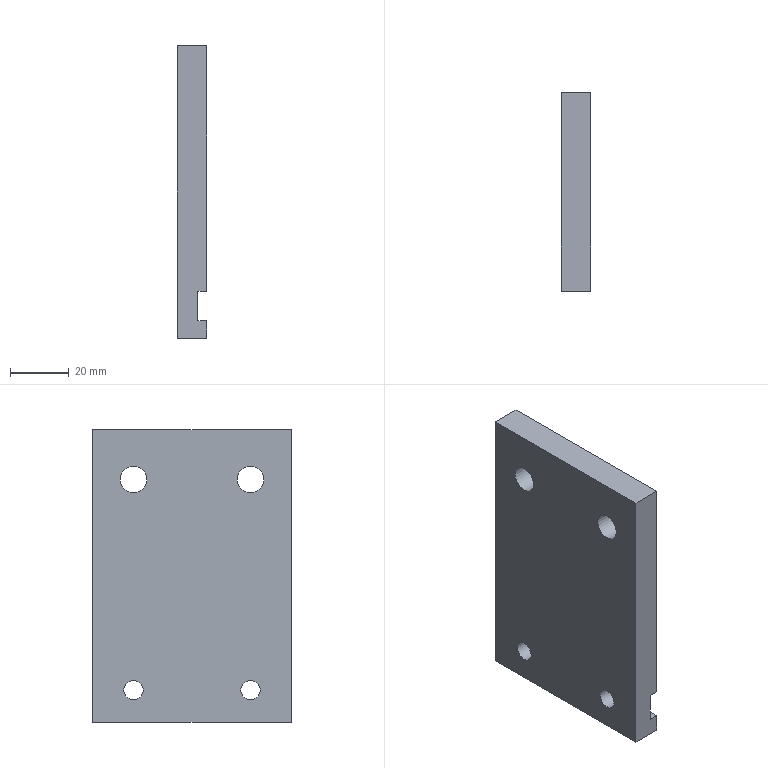Component | NX | GRIPPER_JAW_2 | 1 solid | 14 faces | box 10 x 68 x 100 mm | volume 64209 mm3 | plane 10 | cylinder 4 | commonest cylinder face diameters 6.6 x2 9 x2
STEP:
#1=CARTESIAN_POINT('',(0.,0.,0.));
#2=DIRECTION('',(0.,0.,1.));
#3=DIRECTION('',(1.,0.,0.));
#4=AXIS2_PLACEMENT_3D('',#1,#2,#3);
#5=CARTESIAN_POINT('',(-23.5,223.462,123.766));
#6=VERTEX_POINT('',#5);
#7=CARTESIAN_POINT('',(-23.5,223.462,120.466));
#8=DIRECTION('',(1.,0.,0.));
#9=DIRECTION('',(0.,0.,1.));
#10=AXIS2_PLACEMENT_3D('',#7,#8,#9);
#11=CIRCLE('',#10,3.3);
#12=CARTESIAN_POINT('',(-23.5,223.462,120.466));
#13=DIRECTION('',(1.,0.,0.));
#14=DIRECTION('',(0.,0.,-1.));
#15=AXIS2_PLACEMENT_3D('',#12,#13,#14);
#16=CYLINDRICAL_SURFACE('',#15,3.3);
#17=CARTESIAN_POINT('',(3.142,0.));
#18=DIRECTION('',(1.,0.));
#19=VECTOR('',#18,1.);
#20=LINE('',#17,#19);
#21=(GEOMETRIC_REPRESENTATION_CONTEXT(2)PARAMETRIC_REPRESENTATION_CONTEXT()REPRESENTATION_CONTEXT('',''));
#22=DEFINITIONAL_REPRESENTATION('',(#20),#21);
#23=PCURVE('',#16,#22);
#24=CARTESIAN_POINT('',(-23.5,223.462,192.466));
#25=DIRECTION('',(1.,0.,0.));
#26=DIRECTION('',(0.,0.,-1.));
#27=AXIS2_PLACEMENT_3D('',#24,#25,#26);
#28=PLANE('',#27);
#29=CARTESIAN_POINT('',(72.,0.));
#30=DIRECTION('',(-1.,0.));
#31=AXIS2_PLACEMENT_2D('',#29,#30);
#32=CIRCLE('',#31,3.3);
#33=(GEOMETRIC_REPRESENTATION_CONTEXT(2)PARAMETRIC_REPRESENTATION_CONTEXT()REPRESENTATION_CONTEXT('',''));
#34=DEFINITIONAL_REPRESENTATION('',(#32),#33);
#35=PCURVE('',#28,#34);
#36=SURFACE_CURVE('',#11,(#23,#35),.PCURVE_S1.);
#37=EDGE_CURVE('',#6,#6,#36,.T.);
#38=ORIENTED_EDGE('',*,*,#37,.T.);
#39=CARTESIAN_POINT('',(-16.5,223.462,123.766));
#40=VERTEX_POINT('',#39);
#41=CARTESIAN_POINT('',(-23.5,223.462,123.766));
#42=CARTESIAN_POINT('',(-16.5,223.462,123.766));
#43=B_SPLINE_CURVE_WITH_KNOTS('',1,(#41,#42),.UNSPECIFIED.,.F.,.F.,(2,2),(0.,7.),.PIECEWISE_BEZIER_KNOTS.);
#44=CARTESIAN_POINT('',(9.425,0.));
#45=DIRECTION('',(0.,1.));
#46=VECTOR('',#45,1.);
#47=LINE('',#44,#46);
#48=(GEOMETRIC_REPRESENTATION_CONTEXT(2)PARAMETRIC_REPRESENTATION_CONTEXT()REPRESENTATION_CONTEXT('',''));
#49=DEFINITIONAL_REPRESENTATION('',(#47),#48);
#50=PCURVE('',#16,#49);
#51=CARTESIAN_POINT('',(3.142,0.));
#52=DIRECTION('',(0.,1.));
#53=VECTOR('',#52,1.);
#54=LINE('',#51,#53);
#55=(GEOMETRIC_REPRESENTATION_CONTEXT(2)PARAMETRIC_REPRESENTATION_CONTEXT()REPRESENTATION_CONTEXT('',''));
#56=DEFINITIONAL_REPRESENTATION('',(#54),#55);
#57=PCURVE('',#16,#56);
#58=SEAM_CURVE('',#43,(#50,#57),.PCURVE_S1.);
#59=EDGE_CURVE('',#6,#40,#58,.T.);
#60=ORIENTED_EDGE('',*,*,#59,.T.);
#61=CARTESIAN_POINT('',(-16.5,223.462,120.466));
#62=DIRECTION('',(-1.,0.,0.));
#63=DIRECTION('',(0.,0.,1.));
#64=AXIS2_PLACEMENT_3D('',#61,#62,#63);
#65=CIRCLE('',#64,3.3);
#66=CARTESIAN_POINT('',(9.425,7.));
#67=DIRECTION('',(-1.,0.));
#68=VECTOR('',#67,1.);
#69=LINE('',#66,#68);
#70=(GEOMETRIC_REPRESENTATION_CONTEXT(2)PARAMETRIC_REPRESENTATION_CONTEXT()REPRESENTATION_CONTEXT('',''));
#71=DEFINITIONAL_REPRESENTATION('',(#69),#70);
#72=PCURVE('',#16,#71);
#73=CARTESIAN_POINT('',(-16.5,263.462,120.466));
#74=DIRECTION('',(-1.,0.,0.));
#75=DIRECTION('',(0.,0.,1.));
#76=AXIS2_PLACEMENT_3D('',#73,#74,#75);
#77=PLANE('',#76);
#78=CARTESIAN_POINT('',(0.,-40.));
#79=DIRECTION('',(1.,0.));
#80=AXIS2_PLACEMENT_2D('',#78,#79);
#81=CIRCLE('',#80,3.3);
#82=(GEOMETRIC_REPRESENTATION_CONTEXT(2)PARAMETRIC_REPRESENTATION_CONTEXT()REPRESENTATION_CONTEXT('',''));
#83=DEFINITIONAL_REPRESENTATION('',(#81),#82);
#84=PCURVE('',#77,#83);
#85=SURFACE_CURVE('',#65,(#72,#84),.PCURVE_S1.);
#86=EDGE_CURVE('',#40,#40,#85,.T.);
#87=ORIENTED_EDGE('',*,*,#86,.T.);
#88=ORIENTED_EDGE('',*,*,#59,.F.);
#89=EDGE_LOOP('',(#38,#60,#87,#88));
#90=FACE_BOUND('',#89,.F.);
#91=ADVANCED_FACE('',(#90),#16,.F.);
#92=CARTESIAN_POINT('',(-13.5,209.462,115.466));
#93=VERTEX_POINT('',#92);
#94=CARTESIAN_POINT('',(-13.5,277.462,115.466));
#95=VERTEX_POINT('',#94);
#96=CARTESIAN_POINT('',(-13.5,209.462,115.466));
#97=DIRECTION('',(0.,1.,0.));
#98=VECTOR('',#97,1.);
#99=LINE('',#96,#98);
#100=CARTESIAN_POINT('',(-13.5,223.462,192.466));
#101=DIRECTION('',(1.,0.,0.));
#102=DIRECTION('',(0.,0.,-1.));
#103=AXIS2_PLACEMENT_3D('',#100,#101,#102);
#104=PLANE('',#103);
#105=CARTESIAN_POINT('',(77.,-14.));
#106=DIRECTION('',(0.,1.));
#107=VECTOR('',#106,1.);
#108=LINE('',#105,#107);
#109=(GEOMETRIC_REPRESENTATION_CONTEXT(2)PARAMETRIC_REPRESENTATION_CONTEXT()REPRESENTATION_CONTEXT('',''));
#110=DEFINITIONAL_REPRESENTATION('',(#108),#109);
#111=PCURVE('',#104,#110);
#112=CARTESIAN_POINT('',(-13.5,209.462,115.466));
#113=DIRECTION('',(0.,0.,1.));
#114=DIRECTION('',(1.,0.,0.));
#115=AXIS2_PLACEMENT_3D('',#112,#113,#114);
#116=PLANE('',#115);
#117=CARTESIAN_POINT('',(0.,0.));
#118=DIRECTION('',(0.,1.));
#119=VECTOR('',#118,1.);
#120=LINE('',#117,#119);
#121=(GEOMETRIC_REPRESENTATION_CONTEXT(2)PARAMETRIC_REPRESENTATION_CONTEXT()REPRESENTATION_CONTEXT('',''));
#122=DEFINITIONAL_REPRESENTATION('',(#120),#121);
#123=PCURVE('',#116,#122);
#124=SURFACE_CURVE('',#99,(#111,#123),.PCURVE_S1.);
#125=EDGE_CURVE('',#93,#95,#124,.T.);
#126=ORIENTED_EDGE('',*,*,#125,.F.);
#127=CARTESIAN_POINT('',(-13.5,209.462,109.466));
#128=VERTEX_POINT('',#127);
#129=CARTESIAN_POINT('',(-13.5,209.462,125.466));
#130=DIRECTION('',(0.,0.,1.));
#131=VECTOR('',#130,1.);
#132=LINE('',#129,#131);
#133=CARTESIAN_POINT('',(67.,-14.));
#134=DIRECTION('',(-1.,0.));
#135=VECTOR('',#134,1.);
#136=LINE('',#133,#135);
#137=(GEOMETRIC_REPRESENTATION_CONTEXT(2)PARAMETRIC_REPRESENTATION_CONTEXT()REPRESENTATION_CONTEXT('',''));
#138=DEFINITIONAL_REPRESENTATION('',(#136),#137);
#139=PCURVE('',#104,#138);
#140=CARTESIAN_POINT('',(-23.5,209.462,125.466));
#141=DIRECTION('',(0.,1.,0.));
#142=DIRECTION('',(-1.,0.,0.));
#143=AXIS2_PLACEMENT_3D('',#140,#141,#142);
#144=PLANE('',#143);
#145=CARTESIAN_POINT('',(-10.,0.));
#146=DIRECTION('',(0.,1.));
#147=VECTOR('',#146,1.);
#148=LINE('',#145,#147);
#149=(GEOMETRIC_REPRESENTATION_CONTEXT(2)PARAMETRIC_REPRESENTATION_CONTEXT()REPRESENTATION_CONTEXT('',''));
#150=DEFINITIONAL_REPRESENTATION('',(#148),#149);
#151=PCURVE('',#144,#150);
#152=SURFACE_CURVE('',#132,(#139,#151),.PCURVE_S1.);
#153=EDGE_CURVE('',#128,#93,#152,.T.);
#154=ORIENTED_EDGE('',*,*,#153,.F.);
#155=CARTESIAN_POINT('',(-13.5,277.462,109.466));
#156=VERTEX_POINT('',#155);
#157=CARTESIAN_POINT('',(-13.5,277.462,109.466));
#158=DIRECTION('',(0.,-1.,0.));
#159=VECTOR('',#158,1.);
#160=LINE('',#157,#159);
#161=CARTESIAN_POINT('',(83.,54.));
#162=DIRECTION('',(0.,-1.));
#163=VECTOR('',#162,1.);
#164=LINE('',#161,#163);
#165=(GEOMETRIC_REPRESENTATION_CONTEXT(2)PARAMETRIC_REPRESENTATION_CONTEXT()REPRESENTATION_CONTEXT('',''));
#166=DEFINITIONAL_REPRESENTATION('',(#164),#165);
#167=PCURVE('',#104,#166);
#168=CARTESIAN_POINT('',(-23.5,277.462,109.466));
#169=DIRECTION('',(0.,0.,1.));
#170=DIRECTION('',(1.,0.,0.));
#171=AXIS2_PLACEMENT_3D('',#168,#169,#170);
#172=PLANE('',#171);
#173=CARTESIAN_POINT('',(10.,0.));
#174=DIRECTION('',(0.,-1.));
#175=VECTOR('',#174,1.);
#176=LINE('',#173,#175);
#177=(GEOMETRIC_REPRESENTATION_CONTEXT(2)PARAMETRIC_REPRESENTATION_CONTEXT()REPRESENTATION_CONTEXT('',''));
#178=DEFINITIONAL_REPRESENTATION('',(#176),#177);
#179=PCURVE('',#172,#178);
#180=SURFACE_CURVE('',#160,(#167,#179),.PCURVE_S1.);
#181=EDGE_CURVE('',#156,#128,#180,.T.);
#182=ORIENTED_EDGE('',*,*,#181,.F.);
#183=CARTESIAN_POINT('',(-13.5,277.462,209.466));
#184=DIRECTION('',(0.,0.,-1.));
#185=VECTOR('',#184,1.);
#186=LINE('',#183,#185);
#187=CARTESIAN_POINT('',(-17.,54.));
#188=DIRECTION('',(1.,0.));
#189=VECTOR('',#188,1.);
#190=LINE('',#187,#189);
#191=(GEOMETRIC_REPRESENTATION_CONTEXT(2)PARAMETRIC_REPRESENTATION_CONTEXT()REPRESENTATION_CONTEXT('',''));
#192=DEFINITIONAL_REPRESENTATION('',(#190),#191);
#193=PCURVE('',#104,#192);
#194=CARTESIAN_POINT('',(-23.5,277.462,209.466));
#195=DIRECTION('',(0.,-1.,0.));
#196=DIRECTION('',(1.,0.,0.));
#197=AXIS2_PLACEMENT_3D('',#194,#195,#196);
#198=PLANE('',#197);
#199=CARTESIAN_POINT('',(10.,0.));
#200=DIRECTION('',(0.,-1.));
#201=VECTOR('',#200,1.);
#202=LINE('',#199,#201);
#203=(GEOMETRIC_REPRESENTATION_CONTEXT(2)PARAMETRIC_REPRESENTATION_CONTEXT()REPRESENTATION_CONTEXT('',''));
#204=DEFINITIONAL_REPRESENTATION('',(#202),#203);
#205=PCURVE('',#198,#204);
#206=SURFACE_CURVE('',#186,(#193,#205),.PCURVE_S1.);
#207=EDGE_CURVE('',#95,#156,#206,.T.);
#208=ORIENTED_EDGE('',*,*,#207,.F.);
#209=EDGE_LOOP('',(#126,#154,#182,#208));
#210=FACE_BOUND('',#209,.T.);
#211=ADVANCED_FACE('',(#210),#104,.T.);
#212=ORIENTED_EDGE('',*,*,#181,.T.);
#213=CARTESIAN_POINT('',(-23.5,209.462,109.466));
#214=VERTEX_POINT('',#213);
#215=CARTESIAN_POINT('',(-23.5,209.462,109.466));
#216=DIRECTION('',(1.,0.,0.));
#217=VECTOR('',#216,1.);
#218=LINE('',#215,#217);
#219=CARTESIAN_POINT('',(0.,-68.));
#220=DIRECTION('',(1.,0.));
#221=VECTOR('',#220,1.);
#222=LINE('',#219,#221);
#223=(GEOMETRIC_REPRESENTATION_CONTEXT(2)PARAMETRIC_REPRESENTATION_CONTEXT()REPRESENTATION_CONTEXT('',''));
#224=DEFINITIONAL_REPRESENTATION('',(#222),#223);
#225=PCURVE('',#172,#224);
#226=CARTESIAN_POINT('',(0.,-16.));
#227=DIRECTION('',(-1.,0.));
#228=VECTOR('',#227,1.);
#229=LINE('',#226,#228);
#230=(GEOMETRIC_REPRESENTATION_CONTEXT(2)PARAMETRIC_REPRESENTATION_CONTEXT()REPRESENTATION_CONTEXT('',''));
#231=DEFINITIONAL_REPRESENTATION('',(#229),#230);
#232=PCURVE('',#144,#231);
#233=SURFACE_CURVE('',#218,(#225,#232),.PCURVE_S1.);
#234=EDGE_CURVE('',#214,#128,#233,.T.);
#235=ORIENTED_EDGE('',*,*,#234,.F.);
#236=CARTESIAN_POINT('',(-23.5,277.462,109.466));
#237=VERTEX_POINT('',#236);
#238=CARTESIAN_POINT('',(-23.5,277.462,109.466));
#239=DIRECTION('',(0.,-1.,0.));
#240=VECTOR('',#239,1.);
#241=LINE('',#238,#240);
#242=CARTESIAN_POINT('',(0.,0.));
#243=DIRECTION('',(0.,-1.));
#244=VECTOR('',#243,1.);
#245=LINE('',#242,#244);
#246=(GEOMETRIC_REPRESENTATION_CONTEXT(2)PARAMETRIC_REPRESENTATION_CONTEXT()REPRESENTATION_CONTEXT('',''));
#247=DEFINITIONAL_REPRESENTATION('',(#245),#246);
#248=PCURVE('',#172,#247);
#249=CARTESIAN_POINT('',(83.,54.));
#250=DIRECTION('',(0.,-1.));
#251=VECTOR('',#250,1.);
#252=LINE('',#249,#251);
#253=(GEOMETRIC_REPRESENTATION_CONTEXT(2)PARAMETRIC_REPRESENTATION_CONTEXT()REPRESENTATION_CONTEXT('',''));
#254=DEFINITIONAL_REPRESENTATION('',(#252),#253);
#255=PCURVE('',#28,#254);
#256=SURFACE_CURVE('',#241,(#248,#255),.PCURVE_S1.);
#257=EDGE_CURVE('',#237,#214,#256,.T.);
#258=ORIENTED_EDGE('',*,*,#257,.F.);
#259=CARTESIAN_POINT('',(-23.5,277.462,109.466));
#260=DIRECTION('',(1.,0.,0.));
#261=VECTOR('',#260,1.);
#262=LINE('',#259,#261);
#263=CARTESIAN_POINT('',(0.,0.));
#264=DIRECTION('',(1.,0.));
#265=VECTOR('',#264,1.);
#266=LINE('',#263,#265);
#267=(GEOMETRIC_REPRESENTATION_CONTEXT(2)PARAMETRIC_REPRESENTATION_CONTEXT()REPRESENTATION_CONTEXT('',''));
#268=DEFINITIONAL_REPRESENTATION('',(#266),#267);
#269=PCURVE('',#172,#268);
#270=CARTESIAN_POINT('',(0.,-100.));
#271=DIRECTION('',(1.,0.));
#272=VECTOR('',#271,1.);
#273=LINE('',#270,#272);
#274=(GEOMETRIC_REPRESENTATION_CONTEXT(2)PARAMETRIC_REPRESENTATION_CONTEXT()REPRESENTATION_CONTEXT('',''));
#275=DEFINITIONAL_REPRESENTATION('',(#273),#274);
#276=PCURVE('',#198,#275);
#277=SURFACE_CURVE('',#262,(#269,#276),.PCURVE_S1.);
#278=EDGE_CURVE('',#237,#156,#277,.T.);
#279=ORIENTED_EDGE('',*,*,#278,.T.);
#280=EDGE_LOOP('',(#212,#235,#258,#279));
#281=FACE_BOUND('',#280,.T.);
#282=ADVANCED_FACE('',(#281),#172,.F.);
#283=ORIENTED_EDGE('',*,*,#153,.T.);
#284=CARTESIAN_POINT('',(-16.5,209.462,115.466));
#285=VERTEX_POINT('',#284);
#286=CARTESIAN_POINT('',(-13.5,209.462,115.466));
#287=DIRECTION('',(-1.,0.,0.));
#288=VECTOR('',#287,1.);
#289=LINE('',#286,#288);
#290=CARTESIAN_POINT('',(-10.,-10.));
#291=DIRECTION('',(1.,0.));
#292=VECTOR('',#291,1.);
#293=LINE('',#290,#292);
#294=(GEOMETRIC_REPRESENTATION_CONTEXT(2)PARAMETRIC_REPRESENTATION_CONTEXT()REPRESENTATION_CONTEXT('',''));
#295=DEFINITIONAL_REPRESENTATION('',(#293),#294);
#296=PCURVE('',#144,#295);
#297=CARTESIAN_POINT('',(0.,0.));
#298=DIRECTION('',(-1.,0.));
#299=VECTOR('',#298,1.);
#300=LINE('',#297,#299);
#301=(GEOMETRIC_REPRESENTATION_CONTEXT(2)PARAMETRIC_REPRESENTATION_CONTEXT()REPRESENTATION_CONTEXT('',''));
#302=DEFINITIONAL_REPRESENTATION('',(#300),#301);
#303=PCURVE('',#116,#302);
#304=SURFACE_CURVE('',#289,(#296,#303),.PCURVE_S1.);
#305=EDGE_CURVE('',#93,#285,#304,.T.);
#306=ORIENTED_EDGE('',*,*,#305,.T.);
#307=CARTESIAN_POINT('',(-16.5,209.462,125.466));
#308=VERTEX_POINT('',#307);
#309=CARTESIAN_POINT('',(-16.5,209.462,125.466));
#310=DIRECTION('',(0.,0.,-1.));
#311=VECTOR('',#310,1.);
#312=LINE('',#309,#311);
#313=CARTESIAN_POINT('',(-7.,0.));
#314=DIRECTION('',(0.,-1.));
#315=VECTOR('',#314,1.);
#316=LINE('',#313,#315);
#317=(GEOMETRIC_REPRESENTATION_CONTEXT(2)PARAMETRIC_REPRESENTATION_CONTEXT()REPRESENTATION_CONTEXT('',''));
#318=DEFINITIONAL_REPRESENTATION('',(#316),#317);
#319=PCURVE('',#144,#318);
#320=CARTESIAN_POINT('',(5.,-54.));
#321=DIRECTION('',(-1.,0.));
#322=VECTOR('',#321,1.);
#323=LINE('',#320,#322);
#324=(GEOMETRIC_REPRESENTATION_CONTEXT(2)PARAMETRIC_REPRESENTATION_CONTEXT()REPRESENTATION_CONTEXT('',''));
#325=DEFINITIONAL_REPRESENTATION('',(#323),#324);
#326=PCURVE('',#77,#325);
#327=SURFACE_CURVE('',#312,(#319,#326),.PCURVE_S1.);
#328=EDGE_CURVE('',#308,#285,#327,.T.);
#329=ORIENTED_EDGE('',*,*,#328,.F.);
#330=CARTESIAN_POINT('',(-13.5,209.462,125.466));
#331=VERTEX_POINT('',#330);
#332=CARTESIAN_POINT('',(-13.5,209.462,125.466));
#333=DIRECTION('',(-1.,0.,0.));
#334=VECTOR('',#333,1.);
#335=LINE('',#332,#334);
#336=CARTESIAN_POINT('',(-10.,0.));
#337=DIRECTION('',(1.,0.));
#338=VECTOR('',#337,1.);
#339=LINE('',#336,#338);
#340=(GEOMETRIC_REPRESENTATION_CONTEXT(2)PARAMETRIC_REPRESENTATION_CONTEXT()REPRESENTATION_CONTEXT('',''));
#341=DEFINITIONAL_REPRESENTATION('',(#339),#340);
#342=PCURVE('',#144,#341);
#343=CARTESIAN_POINT('',(-13.5,277.462,125.466));
#344=DIRECTION('',(0.,0.,-1.));
#345=DIRECTION('',(-1.,0.,0.));
#346=AXIS2_PLACEMENT_3D('',#343,#344,#345);
#347=PLANE('',#346);
#348=CARTESIAN_POINT('',(0.,-68.));
#349=DIRECTION('',(1.,0.));
#350=VECTOR('',#349,1.);
#351=LINE('',#348,#350);
#352=(GEOMETRIC_REPRESENTATION_CONTEXT(2)PARAMETRIC_REPRESENTATION_CONTEXT()REPRESENTATION_CONTEXT('',''));
#353=DEFINITIONAL_REPRESENTATION('',(#351),#352);
#354=PCURVE('',#347,#353);
#355=SURFACE_CURVE('',#335,(#342,#354),.PCURVE_S1.);
#356=EDGE_CURVE('',#331,#308,#355,.T.);
#357=ORIENTED_EDGE('',*,*,#356,.F.);
#358=CARTESIAN_POINT('',(-13.5,209.462,209.466));
#359=VERTEX_POINT('',#358);
#360=CARTESIAN_POINT('',(-13.5,209.462,125.466));
#361=DIRECTION('',(0.,0.,1.));
#362=VECTOR('',#361,1.);
#363=LINE('',#360,#362);
#364=CARTESIAN_POINT('',(-10.,0.));
#365=DIRECTION('',(0.,1.));
#366=VECTOR('',#365,1.);
#367=LINE('',#364,#366);
#368=(GEOMETRIC_REPRESENTATION_CONTEXT(2)PARAMETRIC_REPRESENTATION_CONTEXT()REPRESENTATION_CONTEXT('',''));
#369=DEFINITIONAL_REPRESENTATION('',(#367),#368);
#370=PCURVE('',#144,#369);
#371=CARTESIAN_POINT('',(-13.5,223.462,192.466));
#372=DIRECTION('',(1.,0.,0.));
#373=DIRECTION('',(0.,0.,-1.));
#374=AXIS2_PLACEMENT_3D('',#371,#372,#373);
#375=PLANE('',#374);
#376=CARTESIAN_POINT('',(67.,-14.));
#377=DIRECTION('',(-1.,0.));
#378=VECTOR('',#377,1.);
#379=LINE('',#376,#378);
#380=(GEOMETRIC_REPRESENTATION_CONTEXT(2)PARAMETRIC_REPRESENTATION_CONTEXT()REPRESENTATION_CONTEXT('',''));
#381=DEFINITIONAL_REPRESENTATION('',(#379),#380);
#382=PCURVE('',#375,#381);
#383=SURFACE_CURVE('',#363,(#370,#382),.PCURVE_S1.);
#384=EDGE_CURVE('',#331,#359,#383,.T.);
#385=ORIENTED_EDGE('',*,*,#384,.T.);
#386=CARTESIAN_POINT('',(-23.5,209.462,209.466));
#387=VERTEX_POINT('',#386);
#388=CARTESIAN_POINT('',(-23.5,209.462,209.466));
#389=DIRECTION('',(1.,0.,0.));
#390=VECTOR('',#389,1.);
#391=LINE('',#388,#390);
#392=CARTESIAN_POINT('',(0.,84.));
#393=DIRECTION('',(-1.,0.));
#394=VECTOR('',#393,1.);
#395=LINE('',#392,#394);
#396=(GEOMETRIC_REPRESENTATION_CONTEXT(2)PARAMETRIC_REPRESENTATION_CONTEXT()REPRESENTATION_CONTEXT('',''));
#397=DEFINITIONAL_REPRESENTATION('',(#395),#396);
#398=PCURVE('',#144,#397);
#399=CARTESIAN_POINT('',(-23.5,209.462,209.466));
#400=DIRECTION('',(0.,0.,-1.));
#401=DIRECTION('',(-1.,0.,0.));
#402=AXIS2_PLACEMENT_3D('',#399,#400,#401);
#403=PLANE('',#402);
#404=CARTESIAN_POINT('',(0.,0.));
#405=DIRECTION('',(-1.,0.));
#406=VECTOR('',#405,1.);
#407=LINE('',#404,#406);
#408=(GEOMETRIC_REPRESENTATION_CONTEXT(2)PARAMETRIC_REPRESENTATION_CONTEXT()REPRESENTATION_CONTEXT('',''));
#409=DEFINITIONAL_REPRESENTATION('',(#407),#408);
#410=PCURVE('',#403,#409);
#411=SURFACE_CURVE('',#391,(#398,#410),.PCURVE_S1.);
#412=EDGE_CURVE('',#387,#359,#411,.T.);
#413=ORIENTED_EDGE('',*,*,#412,.F.);
#414=CARTESIAN_POINT('',(-23.5,209.462,109.466));
#415=DIRECTION('',(0.,0.,1.));
#416=VECTOR('',#415,1.);
#417=LINE('',#414,#416);
#418=CARTESIAN_POINT('',(0.,-16.));
#419=DIRECTION('',(0.,1.));
#420=VECTOR('',#419,1.);
#421=LINE('',#418,#420);
#422=(GEOMETRIC_REPRESENTATION_CONTEXT(2)PARAMETRIC_REPRESENTATION_CONTEXT()REPRESENTATION_CONTEXT('',''));
#423=DEFINITIONAL_REPRESENTATION('',(#421),#422);
#424=PCURVE('',#144,#423);
#425=CARTESIAN_POINT('',(83.,-14.));
#426=DIRECTION('',(-1.,0.));
#427=VECTOR('',#426,1.);
#428=LINE('',#425,#427);
#429=(GEOMETRIC_REPRESENTATION_CONTEXT(2)PARAMETRIC_REPRESENTATION_CONTEXT()REPRESENTATION_CONTEXT('',''));
#430=DEFINITIONAL_REPRESENTATION('',(#428),#429);
#431=PCURVE('',#28,#430);
#432=SURFACE_CURVE('',#417,(#424,#431),.PCURVE_S1.);
#433=EDGE_CURVE('',#214,#387,#432,.T.);
#434=ORIENTED_EDGE('',*,*,#433,.F.);
#435=ORIENTED_EDGE('',*,*,#234,.T.);
#436=EDGE_LOOP('',(#283,#306,#329,#357,#385,#413,#434,#435));
#437=FACE_BOUND('',#436,.T.);
#438=ADVANCED_FACE('',(#437),#144,.F.);
#439=CARTESIAN_POINT('',(-13.5,277.462,209.466));
#440=VERTEX_POINT('',#439);
#441=CARTESIAN_POINT('',(-13.5,209.462,209.466));
#442=DIRECTION('',(0.,1.,0.));
#443=VECTOR('',#442,1.);
#444=LINE('',#441,#443);
#445=CARTESIAN_POINT('',(-10.,0.));
#446=DIRECTION('',(0.,1.));
#447=VECTOR('',#446,1.);
#448=LINE('',#445,#447);
#449=(GEOMETRIC_REPRESENTATION_CONTEXT(2)PARAMETRIC_REPRESENTATION_CONTEXT()REPRESENTATION_CONTEXT('',''));
#450=DEFINITIONAL_REPRESENTATION('',(#448),#449);
#451=PCURVE('',#403,#450);
#452=CARTESIAN_POINT('',(-17.,-14.));
#453=DIRECTION('',(0.,1.));
#454=VECTOR('',#453,1.);
#455=LINE('',#452,#454);
#456=(GEOMETRIC_REPRESENTATION_CONTEXT(2)PARAMETRIC_REPRESENTATION_CONTEXT()REPRESENTATION_CONTEXT('',''));
#457=DEFINITIONAL_REPRESENTATION('',(#455),#456);
#458=PCURVE('',#375,#457);
#459=SURFACE_CURVE('',#444,(#451,#458),.PCURVE_S1.);
#460=EDGE_CURVE('',#359,#440,#459,.T.);
#461=ORIENTED_EDGE('',*,*,#460,.T.);
#462=CARTESIAN_POINT('',(-23.5,277.462,209.466));
#463=VERTEX_POINT('',#462);
#464=CARTESIAN_POINT('',(-23.5,277.462,209.466));
#465=DIRECTION('',(1.,0.,0.));
#466=VECTOR('',#465,1.);
#467=LINE('',#464,#466);
#468=CARTESIAN_POINT('',(0.,68.));
#469=DIRECTION('',(-1.,0.));
#470=VECTOR('',#469,1.);
#471=LINE('',#468,#470);
#472=(GEOMETRIC_REPRESENTATION_CONTEXT(2)PARAMETRIC_REPRESENTATION_CONTEXT()REPRESENTATION_CONTEXT('',''));
#473=DEFINITIONAL_REPRESENTATION('',(#471),#472);
#474=PCURVE('',#403,#473);
#475=CARTESIAN_POINT('',(0.,0.));
#476=DIRECTION('',(1.,0.));
#477=VECTOR('',#476,1.);
#478=LINE('',#475,#477);
#479=(GEOMETRIC_REPRESENTATION_CONTEXT(2)PARAMETRIC_REPRESENTATION_CONTEXT()REPRESENTATION_CONTEXT('',''));
#480=DEFINITIONAL_REPRESENTATION('',(#478),#479);
#481=PCURVE('',#198,#480);
#482=SURFACE_CURVE('',#467,(#474,#481),.PCURVE_S1.);
#483=EDGE_CURVE('',#463,#440,#482,.T.);
#484=ORIENTED_EDGE('',*,*,#483,.F.);
#485=CARTESIAN_POINT('',(-23.5,209.462,209.466));
#486=DIRECTION('',(0.,1.,0.));
#487=VECTOR('',#486,1.);
#488=LINE('',#485,#487);
#489=CARTESIAN_POINT('',(0.,0.));
#490=DIRECTION('',(0.,1.));
#491=VECTOR('',#490,1.);
#492=LINE('',#489,#491);
#493=(GEOMETRIC_REPRESENTATION_CONTEXT(2)PARAMETRIC_REPRESENTATION_CONTEXT()REPRESENTATION_CONTEXT('',''));
#494=DEFINITIONAL_REPRESENTATION('',(#492),#493);
#495=PCURVE('',#403,#494);
#496=CARTESIAN_POINT('',(-17.,-14.));
#497=DIRECTION('',(0.,1.));
#498=VECTOR('',#497,1.);
#499=LINE('',#496,#498);
#500=(GEOMETRIC_REPRESENTATION_CONTEXT(2)PARAMETRIC_REPRESENTATION_CONTEXT()REPRESENTATION_CONTEXT('',''));
#501=DEFINITIONAL_REPRESENTATION('',(#499),#500);
#502=PCURVE('',#28,#501);
#503=SURFACE_CURVE('',#488,(#495,#502),.PCURVE_S1.);
#504=EDGE_CURVE('',#387,#463,#503,.T.);
#505=ORIENTED_EDGE('',*,*,#504,.F.);
#506=ORIENTED_EDGE('',*,*,#412,.T.);
#507=EDGE_LOOP('',(#461,#484,#505,#506));
#508=FACE_BOUND('',#507,.T.);
#509=ADVANCED_FACE('',(#508),#403,.F.);
#510=CARTESIAN_POINT('',(-16.5,263.462,123.766));
#511=VERTEX_POINT('',#510);
#512=CARTESIAN_POINT('',(-16.5,263.462,120.466));
#513=DIRECTION('',(-1.,0.,0.));
#514=DIRECTION('',(0.,0.,1.));
#515=AXIS2_PLACEMENT_3D('',#512,#513,#514);
#516=CIRCLE('',#515,3.3);
#517=CARTESIAN_POINT('',(-23.5,263.462,120.466));
#518=DIRECTION('',(1.,0.,0.));
#519=DIRECTION('',(0.,0.,-1.));
#520=AXIS2_PLACEMENT_3D('',#517,#518,#519);
#521=CYLINDRICAL_SURFACE('',#520,3.3);
#522=CARTESIAN_POINT('',(9.425,7.));
#523=DIRECTION('',(-1.,0.));
#524=VECTOR('',#523,1.);
#525=LINE('',#522,#524);
#526=(GEOMETRIC_REPRESENTATION_CONTEXT(2)PARAMETRIC_REPRESENTATION_CONTEXT()REPRESENTATION_CONTEXT('',''));
#527=DEFINITIONAL_REPRESENTATION('',(#525),#526);
#528=PCURVE('',#521,#527);
#529=CARTESIAN_POINT('',(0.,0.));
#530=DIRECTION('',(1.,0.));
#531=AXIS2_PLACEMENT_2D('',#529,#530);
#532=CIRCLE('',#531,3.3);
#533=(GEOMETRIC_REPRESENTATION_CONTEXT(2)PARAMETRIC_REPRESENTATION_CONTEXT()REPRESENTATION_CONTEXT('',''));
#534=DEFINITIONAL_REPRESENTATION('',(#532),#533);
#535=PCURVE('',#77,#534);
#536=SURFACE_CURVE('',#516,(#528,#535),.PCURVE_S1.);
#537=EDGE_CURVE('',#511,#511,#536,.T.);
#538=ORIENTED_EDGE('',*,*,#537,.T.);
#539=CARTESIAN_POINT('',(-23.5,263.462,123.766));
#540=VERTEX_POINT('',#539);
#541=CARTESIAN_POINT('',(-23.5,263.462,123.766));
#542=CARTESIAN_POINT('',(-16.5,263.462,123.766));
#543=B_SPLINE_CURVE_WITH_KNOTS('',1,(#541,#542),.UNSPECIFIED.,.F.,.F.,(2,2),(0.,7.),.PIECEWISE_BEZIER_KNOTS.);
#544=CARTESIAN_POINT('',(3.142,0.));
#545=DIRECTION('',(0.,1.));
#546=VECTOR('',#545,1.);
#547=LINE('',#544,#546);
#548=(GEOMETRIC_REPRESENTATION_CONTEXT(2)PARAMETRIC_REPRESENTATION_CONTEXT()REPRESENTATION_CONTEXT('',''));
#549=DEFINITIONAL_REPRESENTATION('',(#547),#548);
#550=PCURVE('',#521,#549);
#551=CARTESIAN_POINT('',(9.425,0.));
#552=DIRECTION('',(0.,1.));
#553=VECTOR('',#552,1.);
#554=LINE('',#551,#553);
#555=(GEOMETRIC_REPRESENTATION_CONTEXT(2)PARAMETRIC_REPRESENTATION_CONTEXT()REPRESENTATION_CONTEXT('',''));
#556=DEFINITIONAL_REPRESENTATION('',(#554),#555);
#557=PCURVE('',#521,#556);
#558=SEAM_CURVE('',#543,(#550,#557),.PCURVE_S1.);
#559=EDGE_CURVE('',#540,#511,#558,.T.);
#560=ORIENTED_EDGE('',*,*,#559,.F.);
#561=CARTESIAN_POINT('',(-23.5,263.462,120.466));
#562=DIRECTION('',(-1.,0.,0.));
#563=DIRECTION('',(0.,0.,1.));
#564=AXIS2_PLACEMENT_3D('',#561,#562,#563);
#565=CIRCLE('',#564,3.3);
#566=CARTESIAN_POINT('',(9.425,0.));
#567=DIRECTION('',(-1.,0.));
#568=VECTOR('',#567,1.);
#569=LINE('',#566,#568);
#570=(GEOMETRIC_REPRESENTATION_CONTEXT(2)PARAMETRIC_REPRESENTATION_CONTEXT()REPRESENTATION_CONTEXT('',''));
#571=DEFINITIONAL_REPRESENTATION('',(#569),#570);
#572=PCURVE('',#521,#571);
#573=CARTESIAN_POINT('',(68.7,40.));
#574=CARTESIAN_POINT('',(68.7,45.716));
#575=CARTESIAN_POINT('',(73.65,42.858));
#576=CARTESIAN_POINT('',(78.6,40.));
#577=CARTESIAN_POINT('',(73.65,37.142));
#578=CARTESIAN_POINT('',(68.7,34.284));
#579=CARTESIAN_POINT('',(68.7,40.));
#580=(BOUNDED_CURVE()B_SPLINE_CURVE(2,(#573,#574,#575,#576,#577,#578,#579),.UNSPECIFIED.,.T.,.F.)B_SPLINE_CURVE_WITH_KNOTS((1,2,2,2,2,1),(-2.094,0.,2.094,4.189,6.283,8.378),.UNSPECIFIED.)CURVE()GEOMETRIC_REPRESENTATION_ITEM()RATIONAL_B_SPLINE_CURVE((1.,0.5,1.,0.5,1.,0.5,1.))REPRESENTATION_ITEM(''));
#581=(GEOMETRIC_REPRESENTATION_CONTEXT(2)PARAMETRIC_REPRESENTATION_CONTEXT()REPRESENTATION_CONTEXT('',''));
#582=DEFINITIONAL_REPRESENTATION('',(#580),#581);
#583=PCURVE('',#28,#582);
#584=SURFACE_CURVE('',#565,(#572,#583),.PCURVE_S1.);
#585=EDGE_CURVE('',#540,#540,#584,.T.);
#586=ORIENTED_EDGE('',*,*,#585,.F.);
#587=ORIENTED_EDGE('',*,*,#559,.T.);
#588=EDGE_LOOP('',(#538,#560,#586,#587));
#589=FACE_BOUND('',#588,.F.);
#590=ADVANCED_FACE('',(#589),#521,.F.);
#591=CARTESIAN_POINT('',(-23.5,223.462,196.966));
#592=VERTEX_POINT('',#591);
#593=CARTESIAN_POINT('',(-23.5,223.462,192.466));
#594=DIRECTION('',(1.,0.,0.));
#595=DIRECTION('',(0.,0.,1.));
#596=AXIS2_PLACEMENT_3D('',#593,#594,#595);
#597=CIRCLE('',#596,4.5);
#598=CARTESIAN_POINT('',(-23.5,223.462,192.466));
#599=DIRECTION('',(1.,0.,0.));
#600=DIRECTION('',(0.,0.,-1.));
#601=AXIS2_PLACEMENT_3D('',#598,#599,#600);
#602=CYLINDRICAL_SURFACE('',#601,4.5);
#603=CARTESIAN_POINT('',(3.142,0.));
#604=DIRECTION('',(1.,0.));
#605=VECTOR('',#604,1.);
#606=LINE('',#603,#605);
#607=(GEOMETRIC_REPRESENTATION_CONTEXT(2)PARAMETRIC_REPRESENTATION_CONTEXT()REPRESENTATION_CONTEXT('',''));
#608=DEFINITIONAL_REPRESENTATION('',(#606),#607);
#609=PCURVE('',#602,#608);
#610=CARTESIAN_POINT('',(0.,0.));
#611=DIRECTION('',(-1.,0.));
#612=AXIS2_PLACEMENT_2D('',#610,#611);
#613=CIRCLE('',#612,4.5);
#614=(GEOMETRIC_REPRESENTATION_CONTEXT(2)PARAMETRIC_REPRESENTATION_CONTEXT()REPRESENTATION_CONTEXT('',''));
#615=DEFINITIONAL_REPRESENTATION('',(#613),#614);
#616=PCURVE('',#28,#615);
#617=SURFACE_CURVE('',#597,(#609,#616),.PCURVE_S1.);
#618=EDGE_CURVE('',#592,#592,#617,.T.);
#619=ORIENTED_EDGE('',*,*,#618,.T.);
#620=CARTESIAN_POINT('',(-13.5,223.462,196.966));
#621=VERTEX_POINT('',#620);
#622=CARTESIAN_POINT('',(-23.5,223.462,196.966));
#623=CARTESIAN_POINT('',(-13.5,223.462,196.966));
#624=B_SPLINE_CURVE_WITH_KNOTS('',1,(#622,#623),.UNSPECIFIED.,.F.,.F.,(2,2),(0.,10.),.PIECEWISE_BEZIER_KNOTS.);
#625=CARTESIAN_POINT('',(9.425,0.));
#626=DIRECTION('',(0.,1.));
#627=VECTOR('',#626,1.);
#628=LINE('',#625,#627);
#629=(GEOMETRIC_REPRESENTATION_CONTEXT(2)PARAMETRIC_REPRESENTATION_CONTEXT()REPRESENTATION_CONTEXT('',''));
#630=DEFINITIONAL_REPRESENTATION('',(#628),#629);
#631=PCURVE('',#602,#630);
#632=CARTESIAN_POINT('',(3.142,0.));
#633=DIRECTION('',(0.,1.));
#634=VECTOR('',#633,1.);
#635=LINE('',#632,#634);
#636=(GEOMETRIC_REPRESENTATION_CONTEXT(2)PARAMETRIC_REPRESENTATION_CONTEXT()REPRESENTATION_CONTEXT('',''));
#637=DEFINITIONAL_REPRESENTATION('',(#635),#636);
#638=PCURVE('',#602,#637);
#639=SEAM_CURVE('',#624,(#631,#638),.PCURVE_S1.);
#640=EDGE_CURVE('',#592,#621,#639,.T.);
#641=ORIENTED_EDGE('',*,*,#640,.T.);
#642=CARTESIAN_POINT('',(-13.5,223.462,192.466));
#643=DIRECTION('',(1.,0.,0.));
#644=DIRECTION('',(0.,0.,1.));
#645=AXIS2_PLACEMENT_3D('',#642,#643,#644);
#646=CIRCLE('',#645,4.5);
#647=CARTESIAN_POINT('',(3.142,10.));
#648=DIRECTION('',(1.,0.));
#649=VECTOR('',#648,1.);
#650=LINE('',#647,#649);
#651=(GEOMETRIC_REPRESENTATION_CONTEXT(2)PARAMETRIC_REPRESENTATION_CONTEXT()REPRESENTATION_CONTEXT('',''));
#652=DEFINITIONAL_REPRESENTATION('',(#650),#651);
#653=PCURVE('',#602,#652);
#654=CARTESIAN_POINT('',(0.,0.));
#655=DIRECTION('',(-1.,0.));
#656=AXIS2_PLACEMENT_2D('',#654,#655);
#657=CIRCLE('',#656,4.5);
#658=(GEOMETRIC_REPRESENTATION_CONTEXT(2)PARAMETRIC_REPRESENTATION_CONTEXT()REPRESENTATION_CONTEXT('',''));
#659=DEFINITIONAL_REPRESENTATION('',(#657),#658);
#660=PCURVE('',#375,#659);
#661=SURFACE_CURVE('',#646,(#653,#660),.PCURVE_S1.);
#662=EDGE_CURVE('',#621,#621,#661,.T.);
#663=ORIENTED_EDGE('',*,*,#662,.F.);
#664=ORIENTED_EDGE('',*,*,#640,.F.);
#665=EDGE_LOOP('',(#619,#641,#663,#664));
#666=FACE_BOUND('',#665,.F.);
#667=ADVANCED_FACE('',(#666),#602,.F.);
#668=CARTESIAN_POINT('',(-13.5,277.462,125.466));
#669=VERTEX_POINT('',#668);
#670=CARTESIAN_POINT('',(-13.5,277.462,209.466));
#671=DIRECTION('',(0.,0.,-1.));
#672=VECTOR('',#671,1.);
#673=LINE('',#670,#672);
#674=CARTESIAN_POINT('',(10.,0.));
#675=DIRECTION('',(0.,-1.));
#676=VECTOR('',#675,1.);
#677=LINE('',#674,#676);
#678=(GEOMETRIC_REPRESENTATION_CONTEXT(2)PARAMETRIC_REPRESENTATION_CONTEXT()REPRESENTATION_CONTEXT('',''));
#679=DEFINITIONAL_REPRESENTATION('',(#677),#678);
#680=PCURVE('',#198,#679);
#681=CARTESIAN_POINT('',(-17.,54.));
#682=DIRECTION('',(1.,0.));
#683=VECTOR('',#682,1.);
#684=LINE('',#681,#683);
#685=(GEOMETRIC_REPRESENTATION_CONTEXT(2)PARAMETRIC_REPRESENTATION_CONTEXT()REPRESENTATION_CONTEXT('',''));
#686=DEFINITIONAL_REPRESENTATION('',(#684),#685);
#687=PCURVE('',#375,#686);
#688=SURFACE_CURVE('',#673,(#680,#687),.PCURVE_S1.);
#689=EDGE_CURVE('',#440,#669,#688,.T.);
#690=ORIENTED_EDGE('',*,*,#689,.T.);
#691=CARTESIAN_POINT('',(-16.5,277.462,125.466));
#692=VERTEX_POINT('',#691);
#693=CARTESIAN_POINT('',(-13.5,277.462,125.466));
#694=DIRECTION('',(-1.,0.,0.));
#695=VECTOR('',#694,1.);
#696=LINE('',#693,#695);
#697=CARTESIAN_POINT('',(10.,-84.));
#698=DIRECTION('',(-1.,0.));
#699=VECTOR('',#698,1.);
#700=LINE('',#697,#699);
#701=(GEOMETRIC_REPRESENTATION_CONTEXT(2)PARAMETRIC_REPRESENTATION_CONTEXT()REPRESENTATION_CONTEXT('',''));
#702=DEFINITIONAL_REPRESENTATION('',(#700),#701);
#703=PCURVE('',#198,#702);
#704=CARTESIAN_POINT('',(0.,0.));
#705=DIRECTION('',(1.,0.));
#706=VECTOR('',#705,1.);
#707=LINE('',#704,#706);
#708=(GEOMETRIC_REPRESENTATION_CONTEXT(2)PARAMETRIC_REPRESENTATION_CONTEXT()REPRESENTATION_CONTEXT('',''));
#709=DEFINITIONAL_REPRESENTATION('',(#707),#708);
#710=PCURVE('',#347,#709);
#711=SURFACE_CURVE('',#696,(#703,#710),.PCURVE_S1.);
#712=EDGE_CURVE('',#669,#692,#711,.T.);
#713=ORIENTED_EDGE('',*,*,#712,.T.);
#714=CARTESIAN_POINT('',(-16.5,277.462,115.466));
#715=VERTEX_POINT('',#714);
#716=CARTESIAN_POINT('',(-16.5,277.462,115.466));
#717=DIRECTION('',(0.,0.,1.));
#718=VECTOR('',#717,1.);
#719=LINE('',#716,#718);
#720=CARTESIAN_POINT('',(7.,-94.));
#721=DIRECTION('',(0.,1.));
#722=VECTOR('',#721,1.);
#723=LINE('',#720,#722);
#724=(GEOMETRIC_REPRESENTATION_CONTEXT(2)PARAMETRIC_REPRESENTATION_CONTEXT()REPRESENTATION_CONTEXT('',''));
#725=DEFINITIONAL_REPRESENTATION('',(#723),#724);
#726=PCURVE('',#198,#725);
#727=CARTESIAN_POINT('',(-5.,14.));
#728=DIRECTION('',(1.,0.));
#729=VECTOR('',#728,1.);
#730=LINE('',#727,#729);
#731=(GEOMETRIC_REPRESENTATION_CONTEXT(2)PARAMETRIC_REPRESENTATION_CONTEXT()REPRESENTATION_CONTEXT('',''));
#732=DEFINITIONAL_REPRESENTATION('',(#730),#731);
#733=PCURVE('',#77,#732);
#734=SURFACE_CURVE('',#719,(#726,#733),.PCURVE_S1.);
#735=EDGE_CURVE('',#715,#692,#734,.T.);
#736=ORIENTED_EDGE('',*,*,#735,.F.);
#737=CARTESIAN_POINT('',(-13.5,277.462,115.466));
#738=DIRECTION('',(-1.,0.,0.));
#739=VECTOR('',#738,1.);
#740=LINE('',#737,#739);
#741=CARTESIAN_POINT('',(10.,-94.));
#742=DIRECTION('',(-1.,0.));
#743=VECTOR('',#742,1.);
#744=LINE('',#741,#743);
#745=(GEOMETRIC_REPRESENTATION_CONTEXT(2)PARAMETRIC_REPRESENTATION_CONTEXT()REPRESENTATION_CONTEXT('',''));
#746=DEFINITIONAL_REPRESENTATION('',(#744),#745);
#747=PCURVE('',#198,#746);
#748=CARTESIAN_POINT('',(0.,68.));
#749=DIRECTION('',(-1.,0.));
#750=VECTOR('',#749,1.);
#751=LINE('',#748,#750);
#752=(GEOMETRIC_REPRESENTATION_CONTEXT(2)PARAMETRIC_REPRESENTATION_CONTEXT()REPRESENTATION_CONTEXT('',''));
#753=DEFINITIONAL_REPRESENTATION('',(#751),#752);
#754=PCURVE('',#116,#753);
#755=SURFACE_CURVE('',#740,(#747,#754),.PCURVE_S1.);
#756=EDGE_CURVE('',#95,#715,#755,.T.);
#757=ORIENTED_EDGE('',*,*,#756,.F.);
#758=ORIENTED_EDGE('',*,*,#207,.T.);
#759=ORIENTED_EDGE('',*,*,#278,.F.);
#760=CARTESIAN_POINT('',(-23.5,277.462,125.466));
#761=DIRECTION('',(0.,0.,-1.));
#762=VECTOR('',#761,1.);
#763=LINE('',#760,#762);
#764=CARTESIAN_POINT('',(0.,-84.));
#765=DIRECTION('',(0.,-1.));
#766=VECTOR('',#765,1.);
#767=LINE('',#764,#766);
#768=(GEOMETRIC_REPRESENTATION_CONTEXT(2)PARAMETRIC_REPRESENTATION_CONTEXT()REPRESENTATION_CONTEXT('',''));
#769=DEFINITIONAL_REPRESENTATION('',(#767),#768);
#770=PCURVE('',#198,#769);
#771=CARTESIAN_POINT('',(67.,54.));
#772=DIRECTION('',(1.,0.));
#773=VECTOR('',#772,1.);
#774=LINE('',#771,#773);
#775=(GEOMETRIC_REPRESENTATION_CONTEXT(2)PARAMETRIC_REPRESENTATION_CONTEXT()REPRESENTATION_CONTEXT('',''));
#776=DEFINITIONAL_REPRESENTATION('',(#774),#775);
#777=PCURVE('',#28,#776);
#778=SURFACE_CURVE('',#763,(#770,#777),.PCURVE_S1.);
#779=EDGE_CURVE('',#463,#237,#778,.T.);
#780=ORIENTED_EDGE('',*,*,#779,.F.);
#781=ORIENTED_EDGE('',*,*,#483,.T.);
#782=EDGE_LOOP('',(#690,#713,#736,#757,#758,#759,#780,#781));
#783=FACE_BOUND('',#782,.T.);
#784=ADVANCED_FACE('',(#783),#198,.F.);
#785=CARTESIAN_POINT('',(-23.5,263.462,196.966));
#786=VERTEX_POINT('',#785);
#787=CARTESIAN_POINT('',(-23.5,263.462,192.466));
#788=DIRECTION('',(-1.,0.,0.));
#789=DIRECTION('',(0.,0.,1.));
#790=AXIS2_PLACEMENT_3D('',#787,#788,#789);
#791=CIRCLE('',#790,4.5);
#792=CARTESIAN_POINT('',(-23.5,263.462,192.466));
#793=DIRECTION('',(1.,0.,0.));
#794=DIRECTION('',(0.,0.,-1.));
#795=AXIS2_PLACEMENT_3D('',#792,#793,#794);
#796=CYLINDRICAL_SURFACE('',#795,4.5);
#797=CARTESIAN_POINT('',(9.425,0.));
#798=DIRECTION('',(-1.,0.));
#799=VECTOR('',#798,1.);
#800=LINE('',#797,#799);
#801=(GEOMETRIC_REPRESENTATION_CONTEXT(2)PARAMETRIC_REPRESENTATION_CONTEXT()REPRESENTATION_CONTEXT('',''));
#802=DEFINITIONAL_REPRESENTATION('',(#800),#801);
#803=PCURVE('',#796,#802);
#804=CARTESIAN_POINT('',(-4.5,40.));
#805=CARTESIAN_POINT('',(-4.5,47.794));
#806=CARTESIAN_POINT('',(2.25,43.897));
#807=CARTESIAN_POINT('',(9.,40.));
#808=CARTESIAN_POINT('',(2.25,36.103));
#809=CARTESIAN_POINT('',(-4.5,32.206));
#810=CARTESIAN_POINT('',(-4.5,40.));
#811=(BOUNDED_CURVE()B_SPLINE_CURVE(2,(#804,#805,#806,#807,#808,#809,#810),.UNSPECIFIED.,.T.,.F.)B_SPLINE_CURVE_WITH_KNOTS((1,2,2,2,2,1),(-2.094,0.,2.094,4.189,6.283,8.378),.UNSPECIFIED.)CURVE()GEOMETRIC_REPRESENTATION_ITEM()RATIONAL_B_SPLINE_CURVE((1.,0.5,1.,0.5,1.,0.5,1.))REPRESENTATION_ITEM(''));
#812=(GEOMETRIC_REPRESENTATION_CONTEXT(2)PARAMETRIC_REPRESENTATION_CONTEXT()REPRESENTATION_CONTEXT('',''));
#813=DEFINITIONAL_REPRESENTATION('',(#811),#812);
#814=PCURVE('',#28,#813);
#815=SURFACE_CURVE('',#791,(#803,#814),.PCURVE_S1.);
#816=EDGE_CURVE('',#786,#786,#815,.T.);
#817=ORIENTED_EDGE('',*,*,#816,.F.);
#818=CARTESIAN_POINT('',(-13.5,263.462,196.966));
#819=VERTEX_POINT('',#818);
#820=CARTESIAN_POINT('',(-23.5,263.462,196.966));
#821=CARTESIAN_POINT('',(-13.5,263.462,196.966));
#822=B_SPLINE_CURVE_WITH_KNOTS('',1,(#820,#821),.UNSPECIFIED.,.F.,.F.,(2,2),(0.,10.),.PIECEWISE_BEZIER_KNOTS.);
#823=CARTESIAN_POINT('',(9.425,0.));
#824=DIRECTION('',(0.,1.));
#825=VECTOR('',#824,1.);
#826=LINE('',#823,#825);
#827=(GEOMETRIC_REPRESENTATION_CONTEXT(2)PARAMETRIC_REPRESENTATION_CONTEXT()REPRESENTATION_CONTEXT('',''));
#828=DEFINITIONAL_REPRESENTATION('',(#826),#827);
#829=PCURVE('',#796,#828);
#830=CARTESIAN_POINT('',(3.142,0.));
#831=DIRECTION('',(0.,1.));
#832=VECTOR('',#831,1.);
#833=LINE('',#830,#832);
#834=(GEOMETRIC_REPRESENTATION_CONTEXT(2)PARAMETRIC_REPRESENTATION_CONTEXT()REPRESENTATION_CONTEXT('',''));
#835=DEFINITIONAL_REPRESENTATION('',(#833),#834);
#836=PCURVE('',#796,#835);
#837=SEAM_CURVE('',#822,(#829,#836),.PCURVE_S1.);
#838=EDGE_CURVE('',#786,#819,#837,.T.);
#839=ORIENTED_EDGE('',*,*,#838,.T.);
#840=CARTESIAN_POINT('',(-13.5,263.462,192.466));
#841=DIRECTION('',(-1.,0.,0.));
#842=DIRECTION('',(0.,0.,1.));
#843=AXIS2_PLACEMENT_3D('',#840,#841,#842);
#844=CIRCLE('',#843,4.5);
#845=CARTESIAN_POINT('',(9.425,10.));
#846=DIRECTION('',(-1.,0.));
#847=VECTOR('',#846,1.);
#848=LINE('',#845,#847);
#849=(GEOMETRIC_REPRESENTATION_CONTEXT(2)PARAMETRIC_REPRESENTATION_CONTEXT()REPRESENTATION_CONTEXT('',''));
#850=DEFINITIONAL_REPRESENTATION('',(#848),#849);
#851=PCURVE('',#796,#850);
#852=CARTESIAN_POINT('',(-4.5,40.));
#853=CARTESIAN_POINT('',(-4.5,47.794));
#854=CARTESIAN_POINT('',(2.25,43.897));
#855=CARTESIAN_POINT('',(9.,40.));
#856=CARTESIAN_POINT('',(2.25,36.103));
#857=CARTESIAN_POINT('',(-4.5,32.206));
#858=CARTESIAN_POINT('',(-4.5,40.));
#859=(BOUNDED_CURVE()B_SPLINE_CURVE(2,(#852,#853,#854,#855,#856,#857,#858),.UNSPECIFIED.,.T.,.F.)B_SPLINE_CURVE_WITH_KNOTS((1,2,2,2,2,1),(-2.094,0.,2.094,4.189,6.283,8.378),.UNSPECIFIED.)CURVE()GEOMETRIC_REPRESENTATION_ITEM()RATIONAL_B_SPLINE_CURVE((1.,0.5,1.,0.5,1.,0.5,1.))REPRESENTATION_ITEM(''));
#860=(GEOMETRIC_REPRESENTATION_CONTEXT(2)PARAMETRIC_REPRESENTATION_CONTEXT()REPRESENTATION_CONTEXT('',''));
#861=DEFINITIONAL_REPRESENTATION('',(#859),#860);
#862=PCURVE('',#375,#861);
#863=SURFACE_CURVE('',#844,(#851,#862),.PCURVE_S1.);
#864=EDGE_CURVE('',#819,#819,#863,.T.);
#865=ORIENTED_EDGE('',*,*,#864,.T.);
#866=ORIENTED_EDGE('',*,*,#838,.F.);
#867=EDGE_LOOP('',(#817,#839,#865,#866));
#868=FACE_BOUND('',#867,.F.);
#869=ADVANCED_FACE('',(#868),#796,.F.);
#870=ORIENTED_EDGE('',*,*,#779,.T.);
#871=ORIENTED_EDGE('',*,*,#257,.T.);
#872=ORIENTED_EDGE('',*,*,#433,.T.);
#873=ORIENTED_EDGE('',*,*,#504,.T.);
#874=EDGE_LOOP('',(#870,#871,#872,#873));
#875=FACE_BOUND('',#874,.T.);
#876=ORIENTED_EDGE('',*,*,#618,.T.);
#877=EDGE_LOOP('',(#876));
#878=FACE_BOUND('',#877,.T.);
#879=ORIENTED_EDGE('',*,*,#585,.F.);
#880=EDGE_LOOP('',(#879));
#881=FACE_BOUND('',#880,.T.);
#882=ORIENTED_EDGE('',*,*,#37,.T.);
#883=EDGE_LOOP('',(#882));
#884=FACE_BOUND('',#883,.T.);
#885=ORIENTED_EDGE('',*,*,#816,.F.);
#886=EDGE_LOOP('',(#885));
#887=FACE_BOUND('',#886,.T.);
#888=ADVANCED_FACE('',(#875,#878,#881,#884,#887),#28,.F.);
#889=CARTESIAN_POINT('',(-13.5,277.462,125.466));
#890=DIRECTION('',(0.,-1.,0.));
#891=VECTOR('',#890,1.);
#892=LINE('',#889,#891);
#893=CARTESIAN_POINT('',(67.,54.));
#894=DIRECTION('',(0.,-1.));
#895=VECTOR('',#894,1.);
#896=LINE('',#893,#895);
#897=(GEOMETRIC_REPRESENTATION_CONTEXT(2)PARAMETRIC_REPRESENTATION_CONTEXT()REPRESENTATION_CONTEXT('',''));
#898=DEFINITIONAL_REPRESENTATION('',(#896),#897);
#899=PCURVE('',#375,#898);
#900=CARTESIAN_POINT('',(0.,0.));
#901=DIRECTION('',(0.,-1.));
#902=VECTOR('',#901,1.);
#903=LINE('',#900,#902);
#904=(GEOMETRIC_REPRESENTATION_CONTEXT(2)PARAMETRIC_REPRESENTATION_CONTEXT()REPRESENTATION_CONTEXT('',''));
#905=DEFINITIONAL_REPRESENTATION('',(#903),#904);
#906=PCURVE('',#347,#905);
#907=SURFACE_CURVE('',#892,(#899,#906),.PCURVE_S1.);
#908=EDGE_CURVE('',#669,#331,#907,.T.);
#909=ORIENTED_EDGE('',*,*,#908,.F.);
#910=ORIENTED_EDGE('',*,*,#689,.F.);
#911=ORIENTED_EDGE('',*,*,#460,.F.);
#912=ORIENTED_EDGE('',*,*,#384,.F.);
#913=EDGE_LOOP('',(#909,#910,#911,#912));
#914=FACE_BOUND('',#913,.T.);
#915=ORIENTED_EDGE('',*,*,#662,.F.);
#916=EDGE_LOOP('',(#915));
#917=FACE_BOUND('',#916,.T.);
#918=ORIENTED_EDGE('',*,*,#864,.T.);
#919=EDGE_LOOP('',(#918));
#920=FACE_BOUND('',#919,.T.);
#921=ADVANCED_FACE('',(#914,#917,#920),#375,.T.);
#922=CARTESIAN_POINT('',(-16.5,209.462,115.466));
#923=DIRECTION('',(0.,-1.,0.));
#924=VECTOR('',#923,1.);
#925=LINE('',#922,#924);
#926=CARTESIAN_POINT('',(-3.,0.));
#927=DIRECTION('',(0.,-1.));
#928=VECTOR('',#927,1.);
#929=LINE('',#926,#928);
#930=(GEOMETRIC_REPRESENTATION_CONTEXT(2)PARAMETRIC_REPRESENTATION_CONTEXT()REPRESENTATION_CONTEXT('',''));
#931=DEFINITIONAL_REPRESENTATION('',(#929),#930);
#932=PCURVE('',#116,#931);
#933=CARTESIAN_POINT('',(-5.,-54.));
#934=DIRECTION('',(0.,-1.));
#935=VECTOR('',#934,1.);
#936=LINE('',#933,#935);
#937=(GEOMETRIC_REPRESENTATION_CONTEXT(2)PARAMETRIC_REPRESENTATION_CONTEXT()REPRESENTATION_CONTEXT('',''));
#938=DEFINITIONAL_REPRESENTATION('',(#936),#937);
#939=PCURVE('',#77,#938);
#940=SURFACE_CURVE('',#925,(#932,#939),.PCURVE_S1.);
#941=EDGE_CURVE('',#715,#285,#940,.T.);
#942=ORIENTED_EDGE('',*,*,#941,.T.);
#943=ORIENTED_EDGE('',*,*,#305,.F.);
#944=ORIENTED_EDGE('',*,*,#125,.T.);
#945=ORIENTED_EDGE('',*,*,#756,.T.);
#946=EDGE_LOOP('',(#942,#943,#944,#945));
#947=FACE_BOUND('',#946,.T.);
#948=ADVANCED_FACE('',(#947),#116,.T.);
#949=CARTESIAN_POINT('',(-16.5,277.462,125.466));
#950=DIRECTION('',(0.,1.,0.));
#951=VECTOR('',#950,1.);
#952=LINE('',#949,#951);
#953=CARTESIAN_POINT('',(3.,0.));
#954=DIRECTION('',(0.,1.));
#955=VECTOR('',#954,1.);
#956=LINE('',#953,#955);
#957=(GEOMETRIC_REPRESENTATION_CONTEXT(2)PARAMETRIC_REPRESENTATION_CONTEXT()REPRESENTATION_CONTEXT('',''));
#958=DEFINITIONAL_REPRESENTATION('',(#956),#957);
#959=PCURVE('',#347,#958);
#960=CARTESIAN_POINT('',(5.,14.));
#961=DIRECTION('',(0.,1.));
#962=VECTOR('',#961,1.);
#963=LINE('',#960,#962);
#964=(GEOMETRIC_REPRESENTATION_CONTEXT(2)PARAMETRIC_REPRESENTATION_CONTEXT()REPRESENTATION_CONTEXT('',''));
#965=DEFINITIONAL_REPRESENTATION('',(#963),#964);
#966=PCURVE('',#77,#965);
#967=SURFACE_CURVE('',#952,(#959,#966),.PCURVE_S1.);
#968=EDGE_CURVE('',#308,#692,#967,.T.);
#969=ORIENTED_EDGE('',*,*,#968,.T.);
#970=ORIENTED_EDGE('',*,*,#712,.F.);
#971=ORIENTED_EDGE('',*,*,#908,.T.);
#972=ORIENTED_EDGE('',*,*,#356,.T.);
#973=EDGE_LOOP('',(#969,#970,#971,#972));
#974=FACE_BOUND('',#973,.T.);
#975=ADVANCED_FACE('',(#974),#347,.T.);
#976=ORIENTED_EDGE('',*,*,#941,.F.);
#977=ORIENTED_EDGE('',*,*,#735,.T.);
#978=ORIENTED_EDGE('',*,*,#968,.F.);
#979=ORIENTED_EDGE('',*,*,#328,.T.);
#980=EDGE_LOOP('',(#976,#977,#978,#979));
#981=FACE_BOUND('',#980,.T.);
#982=ORIENTED_EDGE('',*,*,#537,.T.);
#983=EDGE_LOOP('',(#982));
#984=FACE_BOUND('',#983,.T.);
#985=ORIENTED_EDGE('',*,*,#86,.T.);
#986=EDGE_LOOP('',(#985));
#987=FACE_BOUND('',#986,.T.);
#988=ADVANCED_FACE('',(#981,#984,#987),#77,.F.);
#989=CLOSED_SHELL('',(#91,#211,#282,#438,#509,#590,#667,#784,#869,#888,#921,#948,#975,#988));
#990=MANIFOLD_SOLID_BREP('',#989);
#991=(LENGTH_UNIT()NAMED_UNIT(*)SI_UNIT(.MILLI.,.METRE.));
#992=UNCERTAINTY_MEASURE_WITH_UNIT(LENGTH_MEASURE(0.000002),#991,'','');
#993=(NAMED_UNIT(*)PLANE_ANGLE_UNIT()SI_UNIT($,.RADIAN.));
#994=(NAMED_UNIT(*)SI_UNIT($,.STERADIAN.)SOLID_ANGLE_UNIT());
#995=(GEOMETRIC_REPRESENTATION_CONTEXT(3)GLOBAL_UNCERTAINTY_ASSIGNED_CONTEXT((#992))GLOBAL_UNIT_ASSIGNED_CONTEXT((#991,#993,#994))REPRESENTATION_CONTEXT('',''));
#996=ADVANCED_BREP_SHAPE_REPRESENTATION('',(#4,#990),#995);